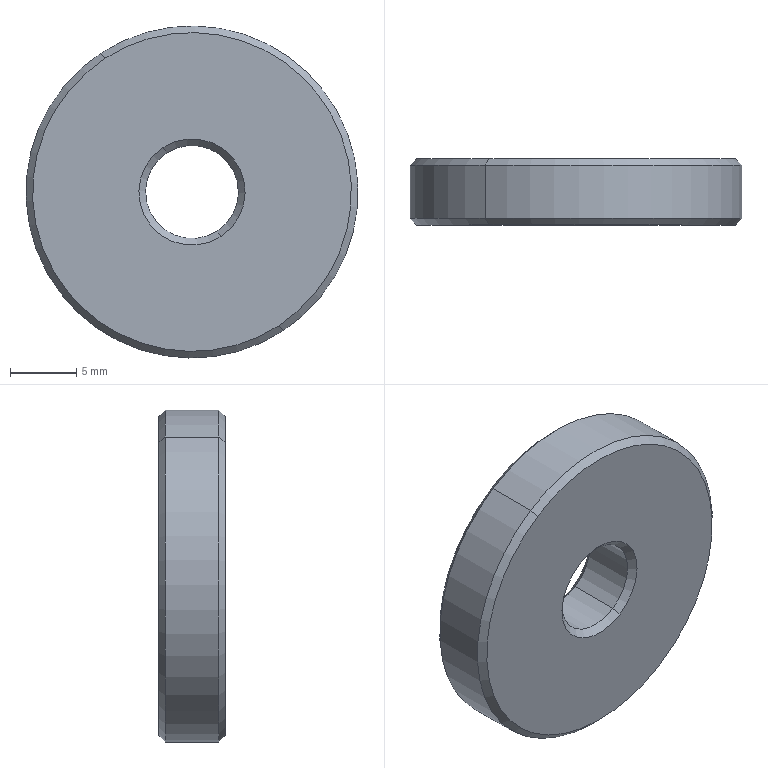Component | SolidWorks | HandwheelEndCap-1 | 1 solid | 14 faces | box 25 x 5 x 25 mm | volume 2237 mm3 | cone 8 | cylinder 4 | plane 2 | commonest cylinder face diameters 7 x2 25 x2
build123d program:
from build123d import *

# Parameters (mm, degrees)
SKETCH1_R           = 12.5
SKETCH1_R_2         = 3.5
BOSS_EXTRUDE1_DEPTH = 5
CHAMFER1_SIZE       = 0.5


with BuildPart() as part:
    # Sketch1 → Boss-Extrude1 (new body)
    with BuildSketch(Plane(origin=(0, 0, 0), x_dir=(1, 0, 0), z_dir=(0, 1, 0))):
        with Locations(Location((0, 0, 0), (0, 0, 270))):
            Circle(SKETCH1_R)
        with Locations(Location((0, 0, 0), (0, 0, 270))):
            Circle(SKETCH1_R_2, mode=Mode.SUBTRACT)
    extrude(amount=BOSS_EXTRUDE1_DEPTH)

    # Chamfer1
    chamfer1_edges = [part.edges().sort_by_distance(p)[0] for p in [
        (0, 0, -12.5),
        (0, 5, -12.5),
        (0, 0, -3.5),
        (0, 5, -3.5),
    ]]
    chamfer(chamfer1_edges, length=CHAMFER1_SIZE)


solid = part.part

# Placed as in the assembly
solid = solid.moved(Location((-29.507, 329.589, 458), (0, 0, 0)))
STEP:
#1=COLOUR_RGB('',0.7922,0.8196,0.9333);
#2=FILL_AREA_STYLE_COLOUR('',#1);
#3=FILL_AREA_STYLE('',(#2));
#4=SURFACE_STYLE_FILL_AREA(#3);
#5=SURFACE_SIDE_STYLE('',(#4));
#6=SURFACE_STYLE_USAGE(.BOTH.,#5);
#7=PRESENTATION_STYLE_ASSIGNMENT((#6));
#8=CARTESIAN_POINT('',(-1.086,12.996,17.916));
#9=VERTEX_POINT('',#8);
#10=CARTESIAN_POINT('',(-1.237,12.996,18.147));
#11=VERTEX_POINT('',#10);
#12=CARTESIAN_POINT('',(-1.162,12.996,18.031));
#13=DIRECTION('',(0.,-1.,0.));
#14=DIRECTION('',(-0.5469,0.,0.8372));
#15=AXIS2_PLACEMENT_3D('',#12,#13,#14);
#16=CIRCLE('',#15,0.1378);
#17=EDGE_CURVE('',#9,#11,#16,.T.);
#18=ORIENTED_EDGE('',*,*,#17,.F.);
#19=CARTESIAN_POINT('',(-1.076,12.976,17.9));
#20=VERTEX_POINT('',#19);
#21=CARTESIAN_POINT('',(-1.086,12.996,17.916));
#22=DIRECTION('',(0.3867,-0.7071,-0.592));
#23=VECTOR('',#22,39.37);
#24=LINE('',#21,#23);
#25=EDGE_CURVE('',#9,#20,#24,.T.);
#26=ORIENTED_EDGE('',*,*,#25,.T.);
#27=CARTESIAN_POINT('',(-1.248,12.976,18.163));
#28=VERTEX_POINT('',#27);
#29=CARTESIAN_POINT('',(-1.162,12.976,18.031));
#30=DIRECTION('',(0.,1.,0.));
#31=DIRECTION('',(-0.5469,0.,0.8372));
#32=AXIS2_PLACEMENT_3D('',#29,#30,#31);
#33=CIRCLE('',#32,0.1575);
#34=EDGE_CURVE('',#28,#20,#33,.T.);
#35=ORIENTED_EDGE('',*,*,#34,.F.);
#36=CARTESIAN_POINT('',(-1.237,12.996,18.147));
#37=DIRECTION('',(-0.3867,-0.7071,0.592));
#38=VECTOR('',#37,39.37);
#39=LINE('',#36,#38);
#40=EDGE_CURVE('',#11,#28,#39,.T.);
#41=ORIENTED_EDGE('',*,*,#40,.F.);
#42=EDGE_LOOP('',(#18,#26,#35,#41));
#43=FACE_OUTER_BOUND('',#42,.T.);
#44=CARTESIAN_POINT('',(-1.162,12.996,18.031));
#45=DIRECTION('',(0.,-1.,0.));
#46=DIRECTION('',(-0.5469,0.,0.8372));
#47=AXIS2_PLACEMENT_3D('',#44,#45,#46);
#48=CONICAL_SURFACE('',#47,0.1378,0.7854);
#49=ADVANCED_FACE('',(#43),#48,.F.);
#50=CARTESIAN_POINT('',(-1.42,12.976,18.427));
#51=VERTEX_POINT('',#50);
#52=CARTESIAN_POINT('',(-0.9033,12.976,17.636));
#53=VERTEX_POINT('',#52);
#54=CARTESIAN_POINT('',(-1.162,12.976,18.031));
#55=DIRECTION('',(0.,-1.,0.));
#56=DIRECTION('',(-0.5469,0.,0.8372));
#57=AXIS2_PLACEMENT_3D('',#54,#55,#56);
#58=CIRCLE('',#57,0.4724);
#59=EDGE_CURVE('',#51,#53,#58,.T.);
#60=ORIENTED_EDGE('',*,*,#59,.F.);
#61=CARTESIAN_POINT('',(-1.431,12.996,18.443));
#62=VERTEX_POINT('',#61);
#63=CARTESIAN_POINT('',(-1.42,12.976,18.427));
#64=DIRECTION('',(-0.3867,0.7071,0.592));
#65=VECTOR('',#64,39.37);
#66=LINE('',#63,#65);
#67=EDGE_CURVE('',#51,#62,#66,.T.);
#68=ORIENTED_EDGE('',*,*,#67,.T.);
#69=CARTESIAN_POINT('',(-0.8925,12.996,17.62));
#70=VERTEX_POINT('',#69);
#71=CARTESIAN_POINT('',(-1.162,12.996,18.031));
#72=DIRECTION('',(0.,1.,0.));
#73=DIRECTION('',(-0.5469,0.,0.8372));
#74=AXIS2_PLACEMENT_3D('',#71,#72,#73);
#75=CIRCLE('',#74,0.4921);
#76=EDGE_CURVE('',#70,#62,#75,.T.);
#77=ORIENTED_EDGE('',*,*,#76,.F.);
#78=CARTESIAN_POINT('',(-0.9033,12.976,17.636));
#79=DIRECTION('',(0.3867,0.7071,-0.592));
#80=VECTOR('',#79,39.37);
#81=LINE('',#78,#80);
#82=EDGE_CURVE('',#53,#70,#81,.T.);
#83=ORIENTED_EDGE('',*,*,#82,.F.);
#84=EDGE_LOOP('',(#60,#68,#77,#83));
#85=FACE_OUTER_BOUND('',#84,.T.);
#86=CARTESIAN_POINT('',(-1.162,12.976,18.031));
#87=DIRECTION('',(0.,1.,0.));
#88=DIRECTION('',(0.5469,0.,-0.8372));
#89=AXIS2_PLACEMENT_3D('',#86,#87,#88);
#90=CONICAL_SURFACE('',#89,0.4724,0.7854);
#91=ADVANCED_FACE('',(#85),#90,.T.);
#92=CARTESIAN_POINT('',(-0.9033,13.173,17.636));
#93=VERTEX_POINT('',#92);
#94=CARTESIAN_POINT('',(-1.42,13.173,18.427));
#95=VERTEX_POINT('',#94);
#96=CARTESIAN_POINT('',(-1.162,13.173,18.031));
#97=DIRECTION('',(0.,1.,0.));
#98=DIRECTION('',(-0.5469,0.,0.8372));
#99=AXIS2_PLACEMENT_3D('',#96,#97,#98);
#100=CIRCLE('',#99,0.4724);
#101=EDGE_CURVE('',#93,#95,#100,.T.);
#102=ORIENTED_EDGE('',*,*,#101,.F.);
#103=CARTESIAN_POINT('',(-0.8925,13.153,17.62));
#104=VERTEX_POINT('',#103);
#105=CARTESIAN_POINT('',(-0.8925,13.153,17.62));
#106=DIRECTION('',(0.3867,-0.7071,-0.592));
#107=VECTOR('',#106,39.37);
#108=LINE('',#105,#107);
#109=EDGE_CURVE('',#93,#104,#108,.T.);
#110=ORIENTED_EDGE('',*,*,#109,.T.);
#111=CARTESIAN_POINT('',(-1.431,13.153,18.443));
#112=VERTEX_POINT('',#111);
#113=CARTESIAN_POINT('',(-1.162,13.153,18.031));
#114=DIRECTION('',(0.,-1.,0.));
#115=DIRECTION('',(-0.5469,0.,0.8372));
#116=AXIS2_PLACEMENT_3D('',#113,#114,#115);
#117=CIRCLE('',#116,0.4921);
#118=EDGE_CURVE('',#112,#104,#117,.T.);
#119=ORIENTED_EDGE('',*,*,#118,.F.);
#120=CARTESIAN_POINT('',(-1.431,13.153,18.443));
#121=DIRECTION('',(-0.3867,-0.7071,0.592));
#122=VECTOR('',#121,39.37);
#123=LINE('',#120,#122);
#124=EDGE_CURVE('',#95,#112,#123,.T.);
#125=ORIENTED_EDGE('',*,*,#124,.F.);
#126=EDGE_LOOP('',(#102,#110,#119,#125));
#127=FACE_OUTER_BOUND('',#126,.T.);
#128=CARTESIAN_POINT('',(-1.162,13.153,18.031));
#129=DIRECTION('',(0.,-1.,0.));
#130=DIRECTION('',(-0.5469,0.,0.8372));
#131=AXIS2_PLACEMENT_3D('',#128,#129,#130);
#132=CONICAL_SURFACE('',#131,0.4921,0.7854);
#133=ADVANCED_FACE('',(#127),#132,.T.);
#134=CARTESIAN_POINT('',(-1.237,13.153,18.147));
#135=VERTEX_POINT('',#134);
#136=CARTESIAN_POINT('',(-1.086,13.153,17.916));
#137=VERTEX_POINT('',#136);
#138=CARTESIAN_POINT('',(-1.162,13.153,18.031));
#139=DIRECTION('',(0.,1.,0.));
#140=DIRECTION('',(-0.5469,0.,0.8372));
#141=AXIS2_PLACEMENT_3D('',#138,#139,#140);
#142=CIRCLE('',#141,0.1378);
#143=EDGE_CURVE('',#135,#137,#142,.T.);
#144=ORIENTED_EDGE('',*,*,#143,.F.);
#145=CARTESIAN_POINT('',(-1.248,13.173,18.163));
#146=VERTEX_POINT('',#145);
#147=CARTESIAN_POINT('',(-1.248,13.173,18.163));
#148=DIRECTION('',(-0.3867,0.7071,0.592));
#149=VECTOR('',#148,39.37);
#150=LINE('',#147,#149);
#151=EDGE_CURVE('',#135,#146,#150,.T.);
#152=ORIENTED_EDGE('',*,*,#151,.T.);
#153=CARTESIAN_POINT('',(-1.076,13.173,17.9));
#154=VERTEX_POINT('',#153);
#155=CARTESIAN_POINT('',(-1.162,13.173,18.031));
#156=DIRECTION('',(0.,-1.,0.));
#157=DIRECTION('',(-0.5469,0.,0.8372));
#158=AXIS2_PLACEMENT_3D('',#155,#156,#157);
#159=CIRCLE('',#158,0.1575);
#160=EDGE_CURVE('',#154,#146,#159,.T.);
#161=ORIENTED_EDGE('',*,*,#160,.F.);
#162=CARTESIAN_POINT('',(-1.076,13.173,17.9));
#163=DIRECTION('',(0.3867,0.7071,-0.592));
#164=VECTOR('',#163,39.37);
#165=LINE('',#162,#164);
#166=EDGE_CURVE('',#137,#154,#165,.T.);
#167=ORIENTED_EDGE('',*,*,#166,.F.);
#168=EDGE_LOOP('',(#144,#152,#161,#167));
#169=FACE_OUTER_BOUND('',#168,.T.);
#170=CARTESIAN_POINT('',(-1.162,13.173,18.031));
#171=DIRECTION('',(0.,1.,0.));
#172=DIRECTION('',(0.5469,0.,-0.8372));
#173=AXIS2_PLACEMENT_3D('',#170,#171,#172);
#174=CONICAL_SURFACE('',#173,0.1575,0.7854);
#175=ADVANCED_FACE('',(#169),#174,.F.);
#176=ORIENTED_EDGE('',*,*,#17,.T.);
#177=CARTESIAN_POINT('',(-1.237,12.976,18.147));
#178=DIRECTION('',(0.,1.,0.));
#179=VECTOR('',#178,39.37);
#180=LINE('',#177,#179);
#181=EDGE_CURVE('',#11,#135,#180,.T.);
#182=ORIENTED_EDGE('',*,*,#181,.T.);
#183=ORIENTED_EDGE('',*,*,#143,.T.);
#184=CARTESIAN_POINT('',(-1.086,12.976,17.916));
#185=DIRECTION('',(0.,1.,0.));
#186=VECTOR('',#185,39.37);
#187=LINE('',#184,#186);
#188=EDGE_CURVE('',#9,#137,#187,.T.);
#189=ORIENTED_EDGE('',*,*,#188,.F.);
#190=EDGE_LOOP('',(#176,#182,#183,#189));
#191=FACE_OUTER_BOUND('',#190,.T.);
#192=CARTESIAN_POINT('',(-1.162,12.976,18.031));
#193=DIRECTION('',(0.,1.,0.));
#194=DIRECTION('',(0.5469,0.,-0.8372));
#195=AXIS2_PLACEMENT_3D('',#192,#193,#194);
#196=CYLINDRICAL_SURFACE('',#195,0.1378);
#197=ADVANCED_FACE('',(#191),#196,.F.);
#198=ORIENTED_EDGE('',*,*,#76,.T.);
#199=CARTESIAN_POINT('',(-1.431,12.976,18.443));
#200=DIRECTION('',(0.,1.,0.));
#201=VECTOR('',#200,39.37);
#202=LINE('',#199,#201);
#203=EDGE_CURVE('',#62,#112,#202,.T.);
#204=ORIENTED_EDGE('',*,*,#203,.T.);
#205=ORIENTED_EDGE('',*,*,#118,.T.);
#206=CARTESIAN_POINT('',(-0.8925,12.976,17.62));
#207=DIRECTION('',(0.,1.,0.));
#208=VECTOR('',#207,39.37);
#209=LINE('',#206,#208);
#210=EDGE_CURVE('',#70,#104,#209,.T.);
#211=ORIENTED_EDGE('',*,*,#210,.F.);
#212=EDGE_LOOP('',(#198,#204,#205,#211));
#213=FACE_OUTER_BOUND('',#212,.T.);
#214=CARTESIAN_POINT('',(-1.162,12.976,18.031));
#215=DIRECTION('',(0.,1.,0.));
#216=DIRECTION('',(0.5469,0.,-0.8372));
#217=AXIS2_PLACEMENT_3D('',#214,#215,#216);
#218=CYLINDRICAL_SURFACE('',#217,0.4921);
#219=ADVANCED_FACE('',(#213),#218,.T.);
#220=CARTESIAN_POINT('',(-1.162,12.976,18.031));
#221=DIRECTION('',(0.,-1.,0.));
#222=DIRECTION('',(-0.5469,0.,0.8372));
#223=AXIS2_PLACEMENT_3D('',#220,#221,#222);
#224=CIRCLE('',#223,0.4724);
#225=EDGE_CURVE('',#53,#51,#224,.T.);
#226=ORIENTED_EDGE('',*,*,#225,.T.);
#227=ORIENTED_EDGE('',*,*,#59,.T.);
#228=EDGE_LOOP('',(#226,#227));
#229=FACE_OUTER_BOUND('',#228,.T.);
#230=ORIENTED_EDGE('',*,*,#34,.T.);
#231=CARTESIAN_POINT('',(-1.162,12.976,18.031));
#232=DIRECTION('',(0.,1.,0.));
#233=DIRECTION('',(-0.5469,0.,0.8372));
#234=AXIS2_PLACEMENT_3D('',#231,#232,#233);
#235=CIRCLE('',#234,0.1575);
#236=EDGE_CURVE('',#20,#28,#235,.T.);
#237=ORIENTED_EDGE('',*,*,#236,.T.);
#238=EDGE_LOOP('',(#230,#237));
#239=FACE_BOUND('',#238,.T.);
#240=CARTESIAN_POINT('',(-1.162,12.976,18.031));
#241=DIRECTION('',(0.,-1.,0.));
#242=DIRECTION('',(-0.5469,0.,0.8372));
#243=AXIS2_PLACEMENT_3D('',#240,#241,#242);
#244=PLANE('',#243);
#245=ADVANCED_FACE('',(#229,#239),#244,.T.);
#246=ORIENTED_EDGE('',*,*,#160,.T.);
#247=CARTESIAN_POINT('',(-1.162,13.173,18.031));
#248=DIRECTION('',(0.,-1.,0.));
#249=DIRECTION('',(-0.5469,0.,0.8372));
#250=AXIS2_PLACEMENT_3D('',#247,#248,#249);
#251=CIRCLE('',#250,0.1575);
#252=EDGE_CURVE('',#146,#154,#251,.T.);
#253=ORIENTED_EDGE('',*,*,#252,.T.);
#254=EDGE_LOOP('',(#246,#253));
#255=FACE_BOUND('',#254,.T.);
#256=CARTESIAN_POINT('',(-1.162,13.173,18.031));
#257=DIRECTION('',(0.,1.,0.));
#258=DIRECTION('',(-0.5469,0.,0.8372));
#259=AXIS2_PLACEMENT_3D('',#256,#257,#258);
#260=CIRCLE('',#259,0.4724);
#261=EDGE_CURVE('',#95,#93,#260,.T.);
#262=ORIENTED_EDGE('',*,*,#261,.T.);
#263=ORIENTED_EDGE('',*,*,#101,.T.);
#264=EDGE_LOOP('',(#262,#263));
#265=FACE_OUTER_BOUND('',#264,.T.);
#266=CARTESIAN_POINT('',(-1.162,13.173,18.031));
#267=DIRECTION('',(0.,-1.,0.));
#268=DIRECTION('',(-0.5469,0.,0.8372));
#269=AXIS2_PLACEMENT_3D('',#266,#267,#268);
#270=PLANE('',#269);
#271=ADVANCED_FACE('',(#255,#265),#270,.F.);
#272=ORIENTED_EDGE('',*,*,#203,.F.);
#273=CARTESIAN_POINT('',(-1.162,12.996,18.031));
#274=DIRECTION('',(0.,1.,0.));
#275=DIRECTION('',(-0.5469,0.,0.8372));
#276=AXIS2_PLACEMENT_3D('',#273,#274,#275);
#277=CIRCLE('',#276,0.4921);
#278=EDGE_CURVE('',#62,#70,#277,.T.);
#279=ORIENTED_EDGE('',*,*,#278,.T.);
#280=ORIENTED_EDGE('',*,*,#210,.T.);
#281=CARTESIAN_POINT('',(-1.162,13.153,18.031));
#282=DIRECTION('',(0.,-1.,0.));
#283=DIRECTION('',(-0.5469,0.,0.8372));
#284=AXIS2_PLACEMENT_3D('',#281,#282,#283);
#285=CIRCLE('',#284,0.4921);
#286=EDGE_CURVE('',#104,#112,#285,.T.);
#287=ORIENTED_EDGE('',*,*,#286,.T.);
#288=EDGE_LOOP('',(#272,#279,#280,#287));
#289=FACE_OUTER_BOUND('',#288,.T.);
#290=CARTESIAN_POINT('',(-1.162,12.976,18.031));
#291=DIRECTION('',(0.,1.,0.));
#292=DIRECTION('',(0.5469,0.,-0.8372));
#293=AXIS2_PLACEMENT_3D('',#290,#291,#292);
#294=CYLINDRICAL_SURFACE('',#293,0.4921);
#295=ADVANCED_FACE('',(#289),#294,.T.);
#296=ORIENTED_EDGE('',*,*,#181,.F.);
#297=CARTESIAN_POINT('',(-1.162,12.996,18.031));
#298=DIRECTION('',(0.,-1.,0.));
#299=DIRECTION('',(-0.5469,0.,0.8372));
#300=AXIS2_PLACEMENT_3D('',#297,#298,#299);
#301=CIRCLE('',#300,0.1378);
#302=EDGE_CURVE('',#11,#9,#301,.T.);
#303=ORIENTED_EDGE('',*,*,#302,.T.);
#304=ORIENTED_EDGE('',*,*,#188,.T.);
#305=CARTESIAN_POINT('',(-1.162,13.153,18.031));
#306=DIRECTION('',(0.,1.,0.));
#307=DIRECTION('',(-0.5469,0.,0.8372));
#308=AXIS2_PLACEMENT_3D('',#305,#306,#307);
#309=CIRCLE('',#308,0.1378);
#310=EDGE_CURVE('',#137,#135,#309,.T.);
#311=ORIENTED_EDGE('',*,*,#310,.T.);
#312=EDGE_LOOP('',(#296,#303,#304,#311));
#313=FACE_OUTER_BOUND('',#312,.T.);
#314=CARTESIAN_POINT('',(-1.162,12.976,18.031));
#315=DIRECTION('',(0.,1.,0.));
#316=DIRECTION('',(0.5469,0.,-0.8372));
#317=AXIS2_PLACEMENT_3D('',#314,#315,#316);
#318=CYLINDRICAL_SURFACE('',#317,0.1378);
#319=ADVANCED_FACE('',(#313),#318,.F.);
#320=ORIENTED_EDGE('',*,*,#151,.F.);
#321=ORIENTED_EDGE('',*,*,#310,.F.);
#322=ORIENTED_EDGE('',*,*,#166,.T.);
#323=ORIENTED_EDGE('',*,*,#252,.F.);
#324=EDGE_LOOP('',(#320,#321,#322,#323));
#325=FACE_OUTER_BOUND('',#324,.T.);
#326=CARTESIAN_POINT('',(-1.162,13.173,18.031));
#327=DIRECTION('',(0.,1.,0.));
#328=DIRECTION('',(0.5469,0.,-0.8372));
#329=AXIS2_PLACEMENT_3D('',#326,#327,#328);
#330=CONICAL_SURFACE('',#329,0.1575,0.7854);
#331=ADVANCED_FACE('',(#325),#330,.F.);
#332=ORIENTED_EDGE('',*,*,#109,.F.);
#333=ORIENTED_EDGE('',*,*,#261,.F.);
#334=ORIENTED_EDGE('',*,*,#124,.T.);
#335=ORIENTED_EDGE('',*,*,#286,.F.);
#336=EDGE_LOOP('',(#332,#333,#334,#335));
#337=FACE_OUTER_BOUND('',#336,.T.);
#338=CARTESIAN_POINT('',(-1.162,13.153,18.031));
#339=DIRECTION('',(0.,-1.,0.));
#340=DIRECTION('',(-0.5469,0.,0.8372));
#341=AXIS2_PLACEMENT_3D('',#338,#339,#340);
#342=CONICAL_SURFACE('',#341,0.4921,0.7854);
#343=ADVANCED_FACE('',(#337),#342,.T.);
#344=ORIENTED_EDGE('',*,*,#67,.F.);
#345=ORIENTED_EDGE('',*,*,#225,.F.);
#346=ORIENTED_EDGE('',*,*,#82,.T.);
#347=ORIENTED_EDGE('',*,*,#278,.F.);
#348=EDGE_LOOP('',(#344,#345,#346,#347));
#349=FACE_OUTER_BOUND('',#348,.T.);
#350=CARTESIAN_POINT('',(-1.162,12.976,18.031));
#351=DIRECTION('',(0.,1.,0.));
#352=DIRECTION('',(0.5469,0.,-0.8372));
#353=AXIS2_PLACEMENT_3D('',#350,#351,#352);
#354=CONICAL_SURFACE('',#353,0.4724,0.7854);
#355=ADVANCED_FACE('',(#349),#354,.T.);
#356=ORIENTED_EDGE('',*,*,#25,.F.);
#357=ORIENTED_EDGE('',*,*,#302,.F.);
#358=ORIENTED_EDGE('',*,*,#40,.T.);
#359=ORIENTED_EDGE('',*,*,#236,.F.);
#360=EDGE_LOOP('',(#356,#357,#358,#359));
#361=FACE_OUTER_BOUND('',#360,.T.);
#362=CARTESIAN_POINT('',(-1.162,12.996,18.031));
#363=DIRECTION('',(0.,-1.,0.));
#364=DIRECTION('',(-0.5469,0.,0.8372));
#365=AXIS2_PLACEMENT_3D('',#362,#363,#364);
#366=CONICAL_SURFACE('',#365,0.1378,0.7854);
#367=ADVANCED_FACE('',(#361),#366,.F.);
#368=CLOSED_SHELL('',(#49,#91,#133,#175,#197,#219,#245,#271,#295,#319,#331,#343,#355,#367));
#369=MANIFOLD_SOLID_BREP('',#368);
#370=STYLED_ITEM('',(#7),#369);
#371=(LENGTH_UNIT()NAMED_UNIT(*)SI_UNIT($,.METRE.));
#372=LENGTH_MEASURE_WITH_UNIT(LENGTH_MEASURE(0.0254),#371);
#373=DIMENSIONAL_EXPONENTS(1.,0.,0.,0.,0.,0.,0.);
#374=(CONVERSION_BASED_UNIT('',#372)LENGTH_UNIT()NAMED_UNIT(#373));
#375=UNCERTAINTY_MEASURE_WITH_UNIT(LENGTH_MEASURE(0.00001),#374,'','');
#376=(NAMED_UNIT(*)PLANE_ANGLE_UNIT()SI_UNIT($,.RADIAN.));
#377=(NAMED_UNIT(*)SI_UNIT($,.STERADIAN.)SOLID_ANGLE_UNIT());
#378=(GEOMETRIC_REPRESENTATION_CONTEXT(3)GLOBAL_UNCERTAINTY_ASSIGNED_CONTEXT((#375))GLOBAL_UNIT_ASSIGNED_CONTEXT((#374,#376,#377))REPRESENTATION_CONTEXT('',''));
#379=MECHANICAL_DESIGN_GEOMETRIC_PRESENTATION_REPRESENTATION('',(#370),#378);
#380=PRESENTATION_LAYER_ASSIGNMENT('','',(#370));
#381=CARTESIAN_POINT('',(0.,0.,0.));
#382=DIRECTION('',(0.,0.,1.));
#383=DIRECTION('',(1.,0.,0.));
#384=AXIS2_PLACEMENT_3D('',#381,#382,#383);
#385=(LENGTH_UNIT()NAMED_UNIT(*)SI_UNIT($,.METRE.));
#386=LENGTH_MEASURE_WITH_UNIT(LENGTH_MEASURE(0.0254),#385);
#387=DIMENSIONAL_EXPONENTS(1.,0.,0.,0.,0.,0.,0.);
#388=(CONVERSION_BASED_UNIT('',#386)LENGTH_UNIT()NAMED_UNIT(#387));
#389=UNCERTAINTY_MEASURE_WITH_UNIT(LENGTH_MEASURE(0.00001),#388,'','');
#390=(NAMED_UNIT(*)PLANE_ANGLE_UNIT()SI_UNIT($,.RADIAN.));
#391=(NAMED_UNIT(*)SI_UNIT($,.STERADIAN.)SOLID_ANGLE_UNIT());
#392=(GEOMETRIC_REPRESENTATION_CONTEXT(3)GLOBAL_UNCERTAINTY_ASSIGNED_CONTEXT((#389))GLOBAL_UNIT_ASSIGNED_CONTEXT((#388,#390,#391))REPRESENTATION_CONTEXT('',''));
#393=ADVANCED_BREP_SHAPE_REPRESENTATION('',(#369,#384),#392);